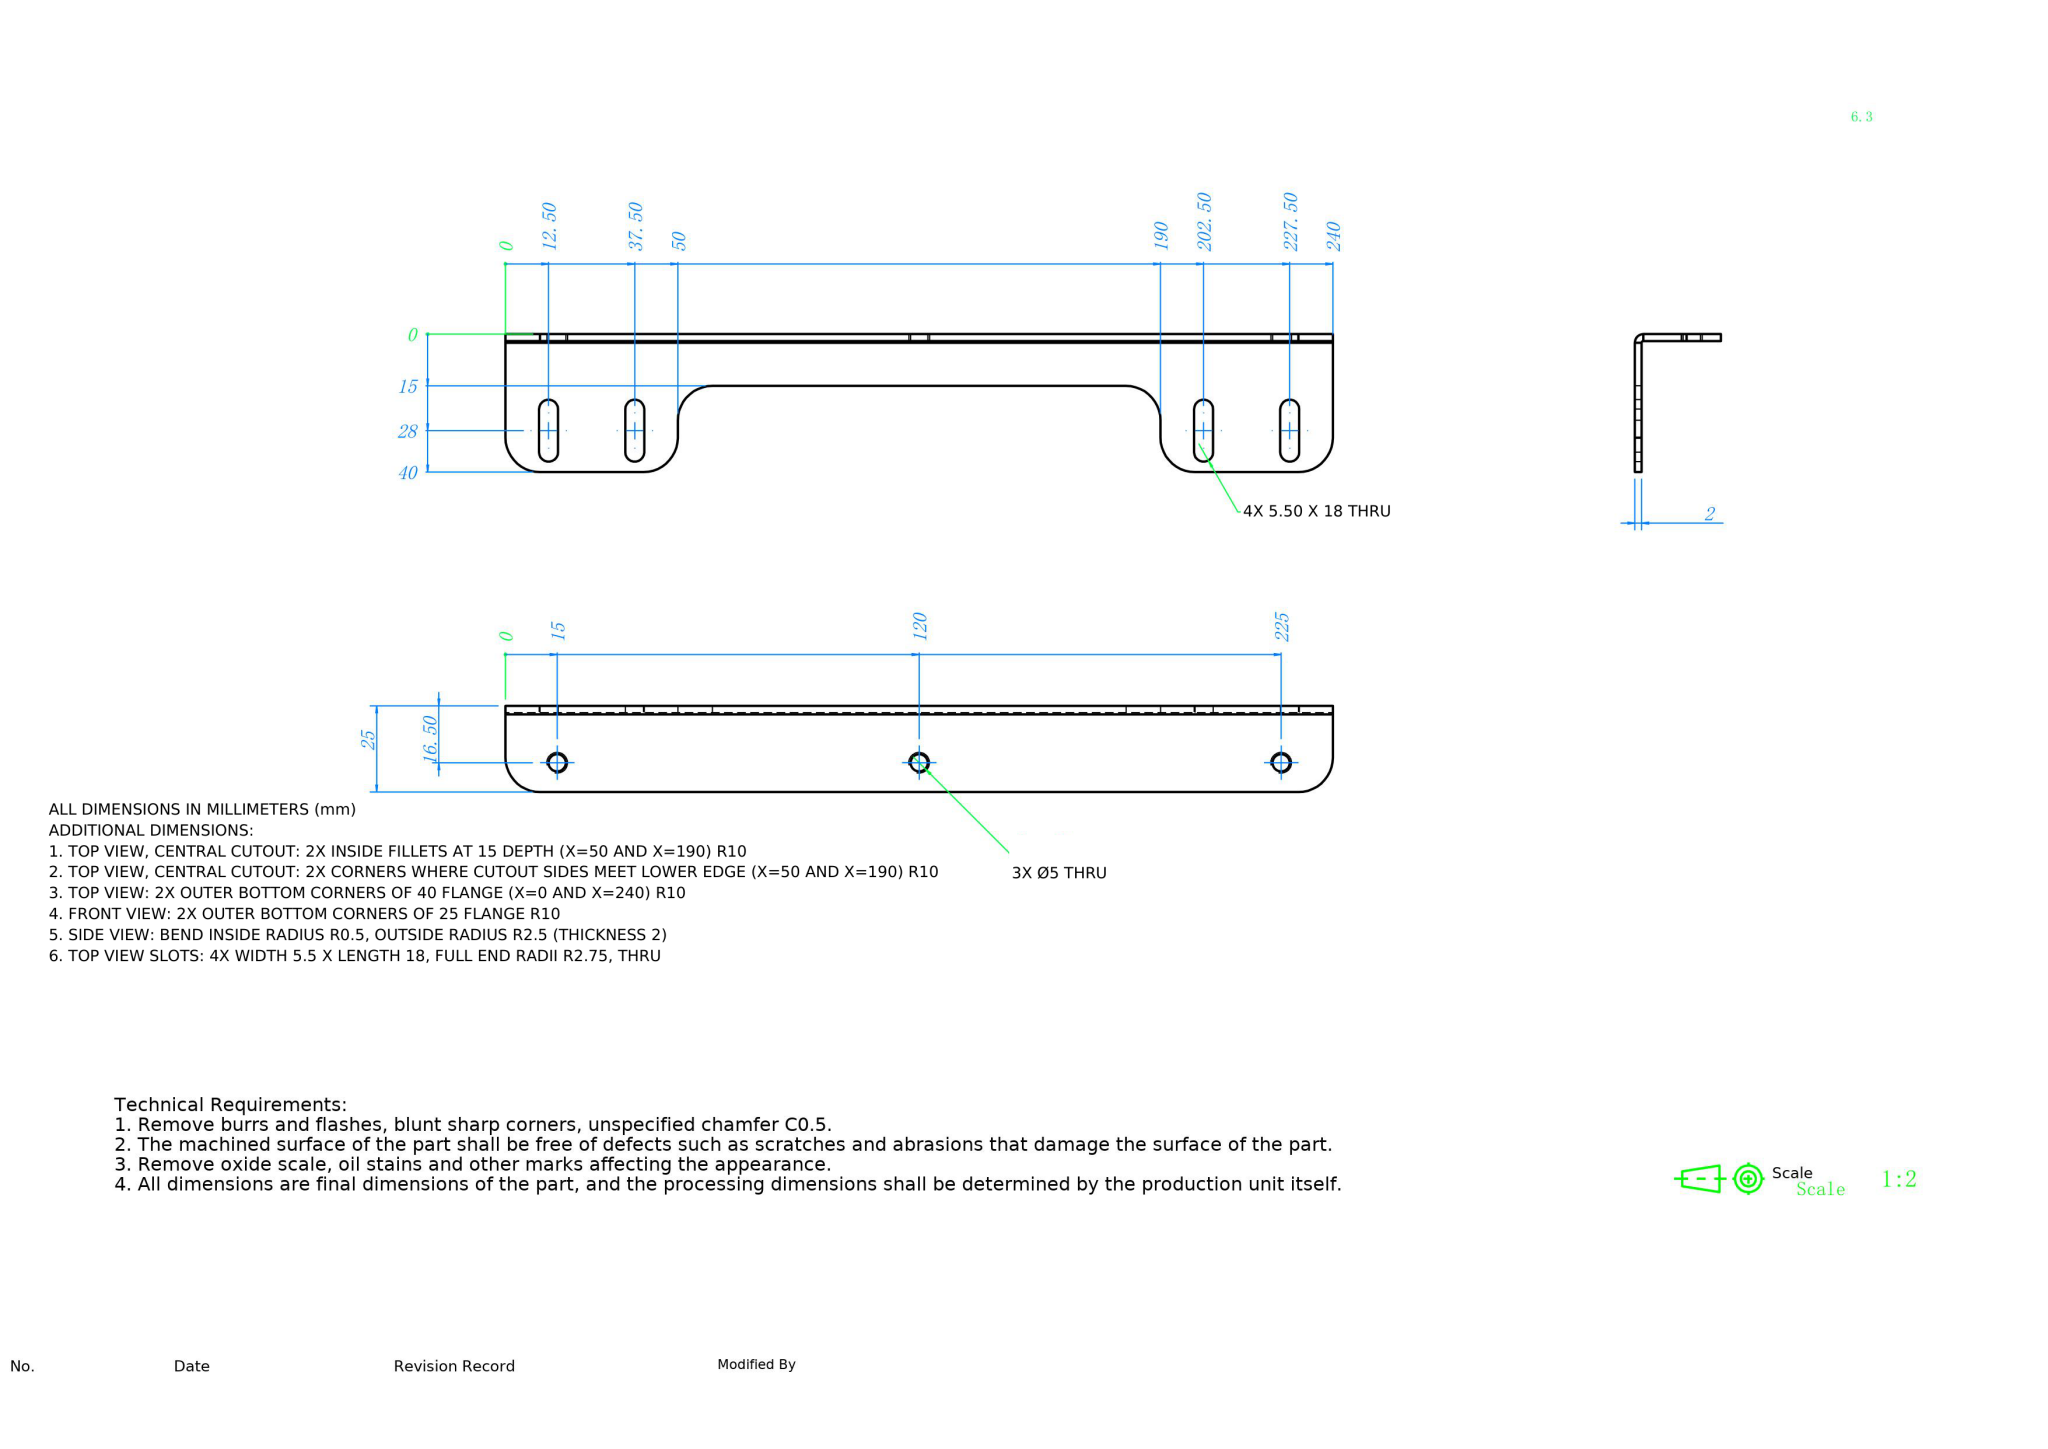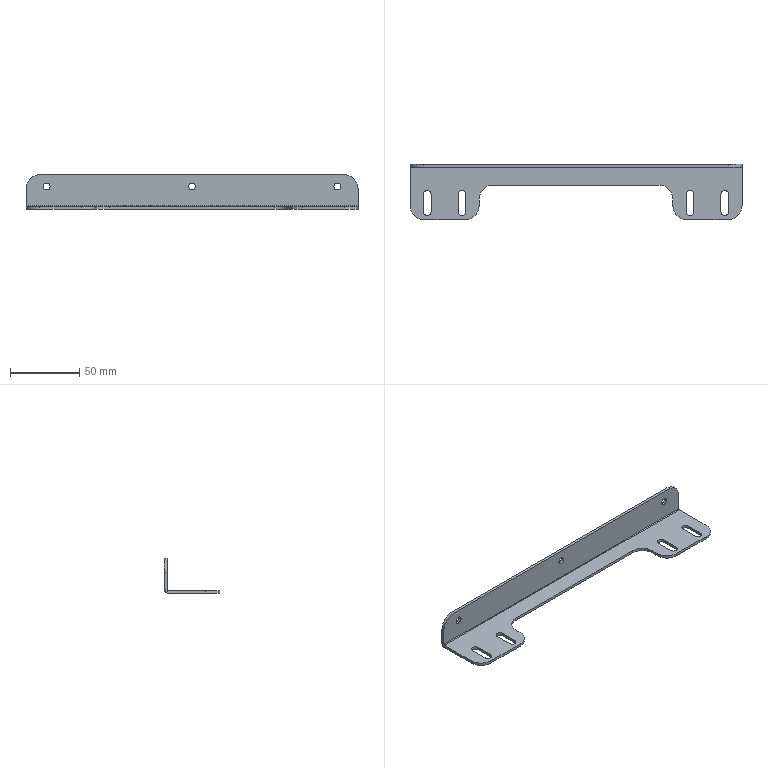Part | NX | mm | 1 solid | 48 faces | box 240 x 40 x 25 mm | volume 21901 mm3 | cylinder 24 | plane 24 | commonest cylinder face diameters 20 x8 5.5 x8 5 x7 1 x1